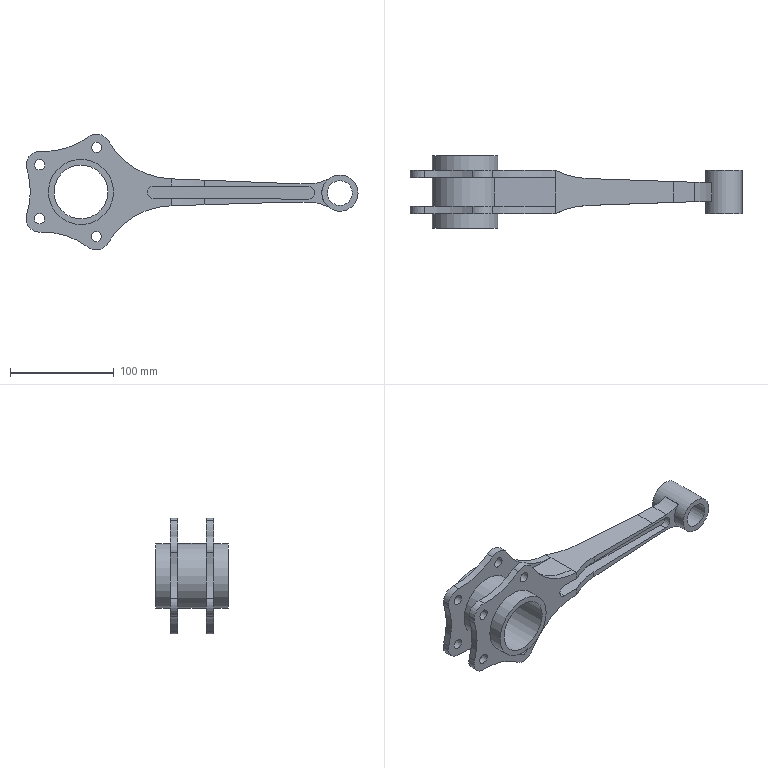Component | NX | MASTER_ROD | 1 solid | 68 faces | volume 257070 mm3 | cylinder 42 | plane 26 | commonest cylinder face diameters 144 x10 26 x8 10 x8 156 x4 12 x4 63 x3 70 x2 52 x1